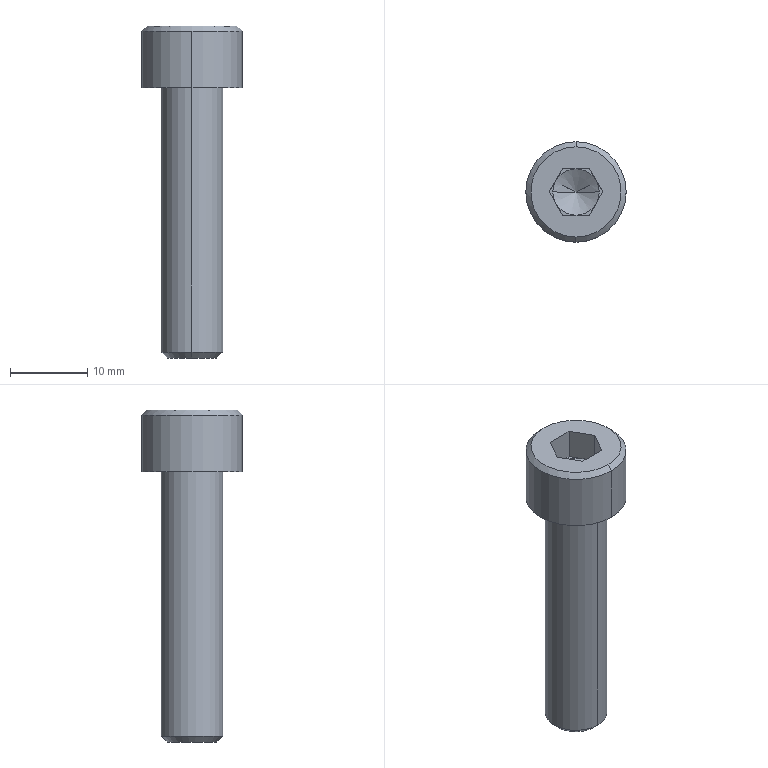Component | SolidWorks | ScrewM8-L35AndSpringWasherAssembly-2_HexSocketHeadCapScrewTAC01-M8-L35(YIHEDA)-1 | 1 solid | 25 faces | box 13 x 13 x 43 mm | volume 2665 mm3 | plane 15 | cone 6 | cylinder 4 | commonest cylinder face diameters 13 x2 8 x2
STEP:
#1=COLOUR_RGB('',0.7922,0.8196,0.9333);
#2=FILL_AREA_STYLE_COLOUR('',#1);
#3=FILL_AREA_STYLE('',(#2));
#4=SURFACE_STYLE_FILL_AREA(#3);
#5=SURFACE_SIDE_STYLE('',(#4));
#6=SURFACE_STYLE_USAGE(.BOTH.,#5);
#7=PRESENTATION_STYLE_ASSIGNMENT((#6));
#8=CARTESIAN_POINT('',(1.489,1.476,0.9883));
#9=VERTEX_POINT('',#8);
#10=CARTESIAN_POINT('',(1.489,1.222,0.9883));
#11=VERTEX_POINT('',#10);
#12=CARTESIAN_POINT('',(1.489,1.349,0.9883));
#13=DIRECTION('',(0.,0.,-1.));
#14=DIRECTION('',(0.,1.,0.));
#15=AXIS2_PLACEMENT_3D('',#12,#13,#14);
#16=CIRCLE('',#15,0.1273);
#17=EDGE_CURVE('',#9,#11,#16,.T.);
#18=ORIENTED_EDGE('',*,*,#17,.F.);
#19=CARTESIAN_POINT('',(1.489,1.507,1.019));
#20=VERTEX_POINT('',#19);
#21=CARTESIAN_POINT('',(1.489,1.507,1.019));
#22=DIRECTION('',(0.,0.7071,0.7071));
#23=VECTOR('',#22,39.37);
#24=LINE('',#21,#23);
#25=EDGE_CURVE('',#9,#20,#24,.T.);
#26=ORIENTED_EDGE('',*,*,#25,.T.);
#27=CARTESIAN_POINT('',(1.489,1.192,1.019));
#28=VERTEX_POINT('',#27);
#29=CARTESIAN_POINT('',(1.489,1.349,1.019));
#30=DIRECTION('',(0.,0.,-1.));
#31=DIRECTION('',(0.,1.,0.));
#32=AXIS2_PLACEMENT_3D('',#29,#30,#31);
#33=CIRCLE('',#32,0.1575);
#34=EDGE_CURVE('',#20,#28,#33,.T.);
#35=ORIENTED_EDGE('',*,*,#34,.T.);
#36=CARTESIAN_POINT('',(1.489,1.192,1.019));
#37=DIRECTION('',(-0.,-0.7071,0.7071));
#38=VECTOR('',#37,39.37);
#39=LINE('',#36,#38);
#40=EDGE_CURVE('',#11,#28,#39,.T.);
#41=ORIENTED_EDGE('',*,*,#40,.F.);
#42=EDGE_LOOP('',(#18,#26,#35,#41));
#43=FACE_OUTER_BOUND('',#42,.T.);
#44=CARTESIAN_POINT('',(1.489,1.349,1.019));
#45=DIRECTION('',(0.,0.,1.));
#46=DIRECTION('',(-0.,-1.,0.));
#47=AXIS2_PLACEMENT_3D('',#44,#45,#46);
#48=CONICAL_SURFACE('',#47,0.1575,0.7854);
#49=ADVANCED_FACE('',(#43),#48,.T.);
#50=CARTESIAN_POINT('',(1.489,1.579,2.681));
#51=VERTEX_POINT('',#50);
#52=CARTESIAN_POINT('',(1.489,1.119,2.681));
#53=VERTEX_POINT('',#52);
#54=CARTESIAN_POINT('',(1.489,1.349,2.681));
#55=DIRECTION('',(0.,0.,-1.));
#56=DIRECTION('',(0.,1.,0.));
#57=AXIS2_PLACEMENT_3D('',#54,#55,#56);
#58=CIRCLE('',#57,0.2303);
#59=EDGE_CURVE('',#51,#53,#58,.T.);
#60=ORIENTED_EDGE('',*,*,#59,.T.);
#61=CARTESIAN_POINT('',(1.489,1.093,2.656));
#62=VERTEX_POINT('',#61);
#63=CARTESIAN_POINT('',(1.489,1.119,2.681));
#64=DIRECTION('',(-0.,-0.7071,-0.7071));
#65=VECTOR('',#64,39.37);
#66=LINE('',#63,#65);
#67=EDGE_CURVE('',#53,#62,#66,.T.);
#68=ORIENTED_EDGE('',*,*,#67,.T.);
#69=CARTESIAN_POINT('',(1.489,1.605,2.656));
#70=VERTEX_POINT('',#69);
#71=CARTESIAN_POINT('',(1.489,1.349,2.656));
#72=DIRECTION('',(0.,0.,-1.));
#73=DIRECTION('',(0.,1.,0.));
#74=AXIS2_PLACEMENT_3D('',#71,#72,#73);
#75=CIRCLE('',#74,0.2559);
#76=EDGE_CURVE('',#70,#62,#75,.T.);
#77=ORIENTED_EDGE('',*,*,#76,.F.);
#78=CARTESIAN_POINT('',(1.489,1.579,2.681));
#79=DIRECTION('',(0.,0.7071,-0.7071));
#80=VECTOR('',#79,39.37);
#81=LINE('',#78,#80);
#82=EDGE_CURVE('',#51,#70,#81,.T.);
#83=ORIENTED_EDGE('',*,*,#82,.F.);
#84=EDGE_LOOP('',(#60,#68,#77,#83));
#85=FACE_OUTER_BOUND('',#84,.T.);
#86=CARTESIAN_POINT('',(1.489,1.349,2.681));
#87=DIRECTION('',(0.,0.,-1.));
#88=DIRECTION('',(0.,1.,0.));
#89=AXIS2_PLACEMENT_3D('',#86,#87,#88);
#90=CONICAL_SURFACE('',#89,0.2303,0.7854);
#91=ADVANCED_FACE('',(#85),#90,.T.);
#92=CARTESIAN_POINT('',(1.489,1.093,2.366));
#93=VERTEX_POINT('',#92);
#94=CARTESIAN_POINT('',(1.489,1.605,2.366));
#95=VERTEX_POINT('',#94);
#96=CARTESIAN_POINT('',(1.489,1.349,2.366));
#97=DIRECTION('',(0.,0.,-1.));
#98=DIRECTION('',(0.,1.,0.));
#99=AXIS2_PLACEMENT_3D('',#96,#97,#98);
#100=CIRCLE('',#99,0.2559);
#101=EDGE_CURVE('',#93,#95,#100,.T.);
#102=ORIENTED_EDGE('',*,*,#101,.F.);
#103=CARTESIAN_POINT('',(1.489,1.093,2.366));
#104=DIRECTION('',(0.,0.,1.));
#105=VECTOR('',#104,39.37);
#106=LINE('',#103,#105);
#107=EDGE_CURVE('',#93,#62,#106,.T.);
#108=ORIENTED_EDGE('',*,*,#107,.T.);
#109=CARTESIAN_POINT('',(1.489,1.349,2.656));
#110=DIRECTION('',(0.,0.,-1.));
#111=DIRECTION('',(0.,1.,0.));
#112=AXIS2_PLACEMENT_3D('',#109,#110,#111);
#113=CIRCLE('',#112,0.2559);
#114=EDGE_CURVE('',#62,#70,#113,.T.);
#115=ORIENTED_EDGE('',*,*,#114,.T.);
#116=CARTESIAN_POINT('',(1.489,1.605,2.366));
#117=DIRECTION('',(0.,0.,1.));
#118=VECTOR('',#117,39.37);
#119=LINE('',#116,#118);
#120=EDGE_CURVE('',#95,#70,#119,.T.);
#121=ORIENTED_EDGE('',*,*,#120,.F.);
#122=EDGE_LOOP('',(#102,#108,#115,#121));
#123=FACE_OUTER_BOUND('',#122,.T.);
#124=CARTESIAN_POINT('',(1.489,1.349,2.366));
#125=DIRECTION('',(0.,0.,1.));
#126=DIRECTION('',(0.,1.,0.));
#127=AXIS2_PLACEMENT_3D('',#124,#125,#126);
#128=CYLINDRICAL_SURFACE('',#127,0.2559);
#129=ADVANCED_FACE('',(#123),#128,.T.);
#130=CARTESIAN_POINT('',(1.489,1.349,2.456));
#131=VERTEX_POINT('',#130);
#132=CARTESIAN_POINT('',(1.371,1.349,2.524));
#133=VERTEX_POINT('',#132);
#134=CARTESIAN_POINT('',(1.371,1.349,2.524));
#135=DIRECTION('',(-0.866,0.,0.5));
#136=VECTOR('',#135,39.37);
#137=LINE('',#134,#136);
#138=EDGE_CURVE('',#131,#133,#137,.T.);
#139=ORIENTED_EDGE('',*,*,#138,.F.);
#140=CARTESIAN_POINT('',(1.607,1.349,2.524));
#141=VERTEX_POINT('',#140);
#142=CARTESIAN_POINT('',(1.607,1.349,2.524));
#143=DIRECTION('',(0.866,-0.,0.5));
#144=VECTOR('',#143,39.37);
#145=LINE('',#142,#144);
#146=EDGE_CURVE('',#131,#141,#145,.T.);
#147=ORIENTED_EDGE('',*,*,#146,.T.);
#148=CARTESIAN_POINT('',(1.592,1.408,2.524));
#149=VERTEX_POINT('',#148);
#150=CARTESIAN_POINT('',(1.489,1.349,2.524));
#151=DIRECTION('',(0.,0.,-1.));
#152=DIRECTION('',(-0.,-1.,0.));
#153=AXIS2_PLACEMENT_3D('',#150,#151,#152);
#154=CIRCLE('',#153,0.1181);
#155=EDGE_CURVE('',#149,#141,#154,.T.);
#156=ORIENTED_EDGE('',*,*,#155,.F.);
#157=CARTESIAN_POINT('',(1.489,1.467,2.524));
#158=VERTEX_POINT('',#157);
#159=CARTESIAN_POINT('',(1.489,1.349,2.524));
#160=DIRECTION('',(0.,0.,-1.));
#161=DIRECTION('',(-0.,-1.,0.));
#162=AXIS2_PLACEMENT_3D('',#159,#160,#161);
#163=CIRCLE('',#162,0.1181);
#164=EDGE_CURVE('',#158,#149,#163,.T.);
#165=ORIENTED_EDGE('',*,*,#164,.F.);
#166=CARTESIAN_POINT('',(1.387,1.408,2.524));
#167=VERTEX_POINT('',#166);
#168=CARTESIAN_POINT('',(1.489,1.349,2.524));
#169=DIRECTION('',(0.,0.,-1.));
#170=DIRECTION('',(-0.,-1.,0.));
#171=AXIS2_PLACEMENT_3D('',#168,#169,#170);
#172=CIRCLE('',#171,0.1181);
#173=EDGE_CURVE('',#167,#158,#172,.T.);
#174=ORIENTED_EDGE('',*,*,#173,.F.);
#175=CARTESIAN_POINT('',(1.489,1.349,2.524));
#176=DIRECTION('',(0.,0.,-1.));
#177=DIRECTION('',(-0.,-1.,0.));
#178=AXIS2_PLACEMENT_3D('',#175,#176,#177);
#179=CIRCLE('',#178,0.1181);
#180=EDGE_CURVE('',#133,#167,#179,.T.);
#181=ORIENTED_EDGE('',*,*,#180,.F.);
#182=EDGE_LOOP('',(#139,#147,#156,#165,#174,#181));
#183=FACE_OUTER_BOUND('',#182,.T.);
#184=CARTESIAN_POINT('',(1.489,1.349,2.524));
#185=DIRECTION('',(0.,-0.,1.));
#186=DIRECTION('',(-1.,0.,0.));
#187=AXIS2_PLACEMENT_3D('',#184,#185,#186);
#188=CONICAL_SURFACE('',#187,0.1181,1.047);
#189=ADVANCED_FACE('',(#183),#188,.F.);
#190=CARTESIAN_POINT('',(1.489,1.349,1.019));
#191=DIRECTION('',(0.,0.,-1.));
#192=DIRECTION('',(0.,1.,0.));
#193=AXIS2_PLACEMENT_3D('',#190,#191,#192);
#194=CIRCLE('',#193,0.1575);
#195=EDGE_CURVE('',#28,#20,#194,.T.);
#196=ORIENTED_EDGE('',*,*,#195,.F.);
#197=CARTESIAN_POINT('',(1.489,1.192,2.366));
#198=VERTEX_POINT('',#197);
#199=CARTESIAN_POINT('',(1.489,1.192,0.9883));
#200=DIRECTION('',(0.,0.,1.));
#201=VECTOR('',#200,39.37);
#202=LINE('',#199,#201);
#203=EDGE_CURVE('',#28,#198,#202,.T.);
#204=ORIENTED_EDGE('',*,*,#203,.T.);
#205=CARTESIAN_POINT('',(1.489,1.507,2.366));
#206=VERTEX_POINT('',#205);
#207=CARTESIAN_POINT('',(1.489,1.349,2.366));
#208=DIRECTION('',(0.,0.,-1.));
#209=DIRECTION('',(0.,1.,0.));
#210=AXIS2_PLACEMENT_3D('',#207,#208,#209);
#211=CIRCLE('',#210,0.1575);
#212=EDGE_CURVE('',#198,#206,#211,.T.);
#213=ORIENTED_EDGE('',*,*,#212,.T.);
#214=CARTESIAN_POINT('',(1.489,1.507,0.9883));
#215=DIRECTION('',(0.,0.,1.));
#216=VECTOR('',#215,39.37);
#217=LINE('',#214,#216);
#218=EDGE_CURVE('',#20,#206,#217,.T.);
#219=ORIENTED_EDGE('',*,*,#218,.F.);
#220=EDGE_LOOP('',(#196,#204,#213,#219));
#221=FACE_OUTER_BOUND('',#220,.T.);
#222=CARTESIAN_POINT('',(1.489,1.349,0.9883));
#223=DIRECTION('',(0.,0.,1.));
#224=DIRECTION('',(0.,1.,0.));
#225=AXIS2_PLACEMENT_3D('',#222,#223,#224);
#226=CYLINDRICAL_SURFACE('',#225,0.1575);
#227=ADVANCED_FACE('',(#221),#226,.T.);
#228=CARTESIAN_POINT('',(1.353,1.349,2.524));
#229=VERTEX_POINT('',#228);
#230=CARTESIAN_POINT('',(1.387,1.29,2.524));
#231=VERTEX_POINT('',#230);
#232=CARTESIAN_POINT('',(1.353,1.349,2.524));
#233=DIRECTION('',(0.5,-0.866,0.));
#234=VECTOR('',#233,39.37);
#235=LINE('',#232,#234);
#236=EDGE_CURVE('',#229,#231,#235,.T.);
#237=ORIENTED_EDGE('',*,*,#236,.T.);
#238=CARTESIAN_POINT('',(1.489,1.349,2.524));
#239=DIRECTION('',(0.,0.,-1.));
#240=DIRECTION('',(-0.,-1.,0.));
#241=AXIS2_PLACEMENT_3D('',#238,#239,#240);
#242=CIRCLE('',#241,0.1181);
#243=EDGE_CURVE('',#231,#133,#242,.T.);
#244=ORIENTED_EDGE('',*,*,#243,.T.);
#245=ORIENTED_EDGE('',*,*,#180,.T.);
#246=CARTESIAN_POINT('',(1.421,1.467,2.524));
#247=DIRECTION('',(-0.5,-0.866,0.));
#248=VECTOR('',#247,39.37);
#249=LINE('',#246,#248);
#250=EDGE_CURVE('',#167,#229,#249,.T.);
#251=ORIENTED_EDGE('',*,*,#250,.T.);
#252=EDGE_LOOP('',(#237,#244,#245,#251));
#253=FACE_OUTER_BOUND('',#252,.T.);
#254=CARTESIAN_POINT('',(1.489,1.349,2.524));
#255=DIRECTION('',(0.,0.,1.));
#256=DIRECTION('',(-0.,-1.,0.));
#257=AXIS2_PLACEMENT_3D('',#254,#255,#256);
#258=PLANE('',#257);
#259=ADVANCED_FACE('',(#253),#258,.T.);
#260=ORIENTED_EDGE('',*,*,#203,.F.);
#261=ORIENTED_EDGE('',*,*,#34,.F.);
#262=ORIENTED_EDGE('',*,*,#218,.T.);
#263=CARTESIAN_POINT('',(1.489,1.349,2.366));
#264=DIRECTION('',(0.,0.,-1.));
#265=DIRECTION('',(0.,1.,0.));
#266=AXIS2_PLACEMENT_3D('',#263,#264,#265);
#267=CIRCLE('',#266,0.1575);
#268=EDGE_CURVE('',#206,#198,#267,.T.);
#269=ORIENTED_EDGE('',*,*,#268,.T.);
#270=EDGE_LOOP('',(#260,#261,#262,#269));
#271=FACE_OUTER_BOUND('',#270,.T.);
#272=CARTESIAN_POINT('',(1.489,1.349,0.9883));
#273=DIRECTION('',(0.,0.,1.));
#274=DIRECTION('',(0.,1.,0.));
#275=AXIS2_PLACEMENT_3D('',#272,#273,#274);
#276=CYLINDRICAL_SURFACE('',#275,0.1575);
#277=ADVANCED_FACE('',(#271),#276,.T.);
#278=ORIENTED_EDGE('',*,*,#146,.F.);
#279=ORIENTED_EDGE('',*,*,#138,.T.);
#280=ORIENTED_EDGE('',*,*,#243,.F.);
#281=CARTESIAN_POINT('',(1.489,1.231,2.524));
#282=VERTEX_POINT('',#281);
#283=CARTESIAN_POINT('',(1.489,1.349,2.524));
#284=DIRECTION('',(0.,0.,-1.));
#285=DIRECTION('',(-0.,-1.,0.));
#286=AXIS2_PLACEMENT_3D('',#283,#284,#285);
#287=CIRCLE('',#286,0.1181);
#288=EDGE_CURVE('',#282,#231,#287,.T.);
#289=ORIENTED_EDGE('',*,*,#288,.F.);
#290=CARTESIAN_POINT('',(1.592,1.29,2.524));
#291=VERTEX_POINT('',#290);
#292=CARTESIAN_POINT('',(1.489,1.349,2.524));
#293=DIRECTION('',(0.,0.,-1.));
#294=DIRECTION('',(-0.,-1.,0.));
#295=AXIS2_PLACEMENT_3D('',#292,#293,#294);
#296=CIRCLE('',#295,0.1181);
#297=EDGE_CURVE('',#291,#282,#296,.T.);
#298=ORIENTED_EDGE('',*,*,#297,.F.);
#299=CARTESIAN_POINT('',(1.489,1.349,2.524));
#300=DIRECTION('',(0.,0.,-1.));
#301=DIRECTION('',(-0.,-1.,0.));
#302=AXIS2_PLACEMENT_3D('',#299,#300,#301);
#303=CIRCLE('',#302,0.1181);
#304=EDGE_CURVE('',#141,#291,#303,.T.);
#305=ORIENTED_EDGE('',*,*,#304,.F.);
#306=EDGE_LOOP('',(#278,#279,#280,#289,#298,#305));
#307=FACE_OUTER_BOUND('',#306,.T.);
#308=CARTESIAN_POINT('',(1.489,1.349,2.524));
#309=DIRECTION('',(0.,-0.,1.));
#310=DIRECTION('',(-1.,0.,0.));
#311=AXIS2_PLACEMENT_3D('',#308,#309,#310);
#312=CONICAL_SURFACE('',#311,0.1181,1.047);
#313=ADVANCED_FACE('',(#307),#312,.F.);
#314=CARTESIAN_POINT('',(1.558,1.467,2.681));
#315=VERTEX_POINT('',#314);
#316=CARTESIAN_POINT('',(1.421,1.467,2.681));
#317=VERTEX_POINT('',#316);
#318=CARTESIAN_POINT('',(1.558,1.467,2.681));
#319=DIRECTION('',(-1.,0.,0.));
#320=VECTOR('',#319,39.37);
#321=LINE('',#318,#320);
#322=EDGE_CURVE('',#315,#317,#321,.T.);
#323=ORIENTED_EDGE('',*,*,#322,.T.);
#324=CARTESIAN_POINT('',(1.421,1.467,2.524));
#325=VERTEX_POINT('',#324);
#326=CARTESIAN_POINT('',(1.421,1.467,2.524));
#327=DIRECTION('',(0.,0.,1.));
#328=VECTOR('',#327,39.37);
#329=LINE('',#326,#328);
#330=EDGE_CURVE('',#325,#317,#329,.T.);
#331=ORIENTED_EDGE('',*,*,#330,.F.);
#332=CARTESIAN_POINT('',(1.558,1.467,2.524));
#333=DIRECTION('',(-1.,0.,0.));
#334=VECTOR('',#333,39.37);
#335=LINE('',#332,#334);
#336=EDGE_CURVE('',#158,#325,#335,.T.);
#337=ORIENTED_EDGE('',*,*,#336,.F.);
#338=CARTESIAN_POINT('',(1.558,1.467,2.524));
#339=VERTEX_POINT('',#338);
#340=CARTESIAN_POINT('',(1.558,1.467,2.524));
#341=DIRECTION('',(-1.,0.,0.));
#342=VECTOR('',#341,39.37);
#343=LINE('',#340,#342);
#344=EDGE_CURVE('',#339,#158,#343,.T.);
#345=ORIENTED_EDGE('',*,*,#344,.F.);
#346=CARTESIAN_POINT('',(1.558,1.467,2.524));
#347=DIRECTION('',(0.,0.,1.));
#348=VECTOR('',#347,39.37);
#349=LINE('',#346,#348);
#350=EDGE_CURVE('',#339,#315,#349,.T.);
#351=ORIENTED_EDGE('',*,*,#350,.T.);
#352=EDGE_LOOP('',(#323,#331,#337,#345,#351));
#353=FACE_OUTER_BOUND('',#352,.T.);
#354=CARTESIAN_POINT('',(1.558,1.467,2.524));
#355=DIRECTION('',(0.,1.,0.));
#356=DIRECTION('',(0.,0.,1.));
#357=AXIS2_PLACEMENT_3D('',#354,#355,#356);
#358=PLANE('',#357);
#359=ADVANCED_FACE('',(#353),#358,.F.);
#360=CARTESIAN_POINT('',(1.558,1.231,2.681));
#361=VERTEX_POINT('',#360);
#362=CARTESIAN_POINT('',(1.626,1.349,2.681));
#363=VERTEX_POINT('',#362);
#364=CARTESIAN_POINT('',(1.558,1.231,2.681));
#365=DIRECTION('',(0.5,0.866,0.));
#366=VECTOR('',#365,39.37);
#367=LINE('',#364,#366);
#368=EDGE_CURVE('',#361,#363,#367,.T.);
#369=ORIENTED_EDGE('',*,*,#368,.T.);
#370=CARTESIAN_POINT('',(1.626,1.349,2.524));
#371=VERTEX_POINT('',#370);
#372=CARTESIAN_POINT('',(1.626,1.349,2.524));
#373=DIRECTION('',(0.,0.,1.));
#374=VECTOR('',#373,39.37);
#375=LINE('',#372,#374);
#376=EDGE_CURVE('',#371,#363,#375,.T.);
#377=ORIENTED_EDGE('',*,*,#376,.F.);
#378=CARTESIAN_POINT('',(1.558,1.231,2.524));
#379=DIRECTION('',(0.5,0.866,0.));
#380=VECTOR('',#379,39.37);
#381=LINE('',#378,#380);
#382=EDGE_CURVE('',#291,#371,#381,.T.);
#383=ORIENTED_EDGE('',*,*,#382,.F.);
#384=CARTESIAN_POINT('',(1.558,1.231,2.524));
#385=VERTEX_POINT('',#384);
#386=CARTESIAN_POINT('',(1.558,1.231,2.524));
#387=DIRECTION('',(0.5,0.866,0.));
#388=VECTOR('',#387,39.37);
#389=LINE('',#386,#388);
#390=EDGE_CURVE('',#385,#291,#389,.T.);
#391=ORIENTED_EDGE('',*,*,#390,.F.);
#392=CARTESIAN_POINT('',(1.558,1.231,2.524));
#393=DIRECTION('',(0.,0.,1.));
#394=VECTOR('',#393,39.37);
#395=LINE('',#392,#394);
#396=EDGE_CURVE('',#385,#361,#395,.T.);
#397=ORIENTED_EDGE('',*,*,#396,.T.);
#398=EDGE_LOOP('',(#369,#377,#383,#391,#397));
#399=FACE_OUTER_BOUND('',#398,.T.);
#400=CARTESIAN_POINT('',(1.558,1.231,2.524));
#401=DIRECTION('',(0.866,-0.5,0.));
#402=DIRECTION('',(0.,0.,-1.));
#403=AXIS2_PLACEMENT_3D('',#400,#401,#402);
#404=PLANE('',#403);
#405=ADVANCED_FACE('',(#399),#404,.F.);
#406=ORIENTED_EDGE('',*,*,#390,.T.);
#407=ORIENTED_EDGE('',*,*,#297,.T.);
#408=CARTESIAN_POINT('',(1.421,1.231,2.524));
#409=DIRECTION('',(1.,-0.,0.));
#410=VECTOR('',#409,39.37);
#411=LINE('',#408,#410);
#412=EDGE_CURVE('',#282,#385,#411,.T.);
#413=ORIENTED_EDGE('',*,*,#412,.T.);
#414=EDGE_LOOP('',(#406,#407,#413));
#415=FACE_OUTER_BOUND('',#414,.T.);
#416=CARTESIAN_POINT('',(1.489,1.349,2.524));
#417=DIRECTION('',(0.,0.,1.));
#418=DIRECTION('',(-0.,-1.,0.));
#419=AXIS2_PLACEMENT_3D('',#416,#417,#418);
#420=PLANE('',#419);
#421=ADVANCED_FACE('',(#415),#420,.T.);
#422=CARTESIAN_POINT('',(1.489,1.349,2.366));
#423=DIRECTION('',(0.,0.,-1.));
#424=DIRECTION('',(0.,1.,0.));
#425=AXIS2_PLACEMENT_3D('',#422,#423,#424);
#426=CIRCLE('',#425,0.2559);
#427=EDGE_CURVE('',#95,#93,#426,.T.);
#428=ORIENTED_EDGE('',*,*,#427,.T.);
#429=ORIENTED_EDGE('',*,*,#101,.T.);
#430=EDGE_LOOP('',(#428,#429));
#431=FACE_OUTER_BOUND('',#430,.T.);
#432=ORIENTED_EDGE('',*,*,#268,.F.);
#433=ORIENTED_EDGE('',*,*,#212,.F.);
#434=EDGE_LOOP('',(#432,#433));
#435=FACE_BOUND('',#434,.T.);
#436=CARTESIAN_POINT('',(1.745,1.349,2.366));
#437=DIRECTION('',(0.,0.,1.));
#438=DIRECTION('',(-0.,-1.,0.));
#439=AXIS2_PLACEMENT_3D('',#436,#437,#438);
#440=PLANE('',#439);
#441=ADVANCED_FACE('',(#431,#435),#440,.F.);
#442=ORIENTED_EDGE('',*,*,#59,.F.);
#443=CARTESIAN_POINT('',(1.489,1.349,2.681));
#444=DIRECTION('',(0.,0.,-1.));
#445=DIRECTION('',(0.,1.,0.));
#446=AXIS2_PLACEMENT_3D('',#443,#444,#445);
#447=CIRCLE('',#446,0.2303);
#448=EDGE_CURVE('',#53,#51,#447,.T.);
#449=ORIENTED_EDGE('',*,*,#448,.F.);
#450=EDGE_LOOP('',(#442,#449));
#451=FACE_OUTER_BOUND('',#450,.T.);
#452=CARTESIAN_POINT('',(1.353,1.349,2.681));
#453=VERTEX_POINT('',#452);
#454=CARTESIAN_POINT('',(1.421,1.231,2.681));
#455=VERTEX_POINT('',#454);
#456=CARTESIAN_POINT('',(1.353,1.349,2.681));
#457=DIRECTION('',(0.5,-0.866,0.));
#458=VECTOR('',#457,39.37);
#459=LINE('',#456,#458);
#460=EDGE_CURVE('',#453,#455,#459,.T.);
#461=ORIENTED_EDGE('',*,*,#460,.F.);
#462=CARTESIAN_POINT('',(1.421,1.467,2.681));
#463=DIRECTION('',(-0.5,-0.866,0.));
#464=VECTOR('',#463,39.37);
#465=LINE('',#462,#464);
#466=EDGE_CURVE('',#317,#453,#465,.T.);
#467=ORIENTED_EDGE('',*,*,#466,.F.);
#468=ORIENTED_EDGE('',*,*,#322,.F.);
#469=CARTESIAN_POINT('',(1.626,1.349,2.681));
#470=DIRECTION('',(-0.5,0.866,0.));
#471=VECTOR('',#470,39.37);
#472=LINE('',#469,#471);
#473=EDGE_CURVE('',#363,#315,#472,.T.);
#474=ORIENTED_EDGE('',*,*,#473,.F.);
#475=ORIENTED_EDGE('',*,*,#368,.F.);
#476=CARTESIAN_POINT('',(1.421,1.231,2.681));
#477=DIRECTION('',(1.,-0.,0.));
#478=VECTOR('',#477,39.37);
#479=LINE('',#476,#478);
#480=EDGE_CURVE('',#455,#361,#479,.T.);
#481=ORIENTED_EDGE('',*,*,#480,.F.);
#482=EDGE_LOOP('',(#461,#467,#468,#474,#475,#481));
#483=FACE_BOUND('',#482,.T.);
#484=CARTESIAN_POINT('',(1.489,1.349,2.681));
#485=DIRECTION('',(0.,0.,-1.));
#486=DIRECTION('',(-1.,0.,0.));
#487=AXIS2_PLACEMENT_3D('',#484,#485,#486);
#488=PLANE('',#487);
#489=ADVANCED_FACE('',(#451,#483),#488,.F.);
#490=CARTESIAN_POINT('',(1.489,1.349,0.9883));
#491=DIRECTION('',(0.,0.,-1.));
#492=DIRECTION('',(0.,1.,0.));
#493=AXIS2_PLACEMENT_3D('',#490,#491,#492);
#494=CIRCLE('',#493,0.1273);
#495=EDGE_CURVE('',#11,#9,#494,.T.);
#496=ORIENTED_EDGE('',*,*,#495,.T.);
#497=ORIENTED_EDGE('',*,*,#17,.T.);
#498=EDGE_LOOP('',(#496,#497));
#499=FACE_OUTER_BOUND('',#498,.T.);
#500=CARTESIAN_POINT('',(1.617,1.349,0.9883));
#501=DIRECTION('',(0.,0.,1.));
#502=DIRECTION('',(-0.,-1.,0.));
#503=AXIS2_PLACEMENT_3D('',#500,#501,#502);
#504=PLANE('',#503);
#505=ADVANCED_FACE('',(#499),#504,.F.);
#506=ORIENTED_EDGE('',*,*,#107,.F.);
#507=ORIENTED_EDGE('',*,*,#427,.F.);
#508=ORIENTED_EDGE('',*,*,#120,.T.);
#509=ORIENTED_EDGE('',*,*,#76,.T.);
#510=EDGE_LOOP('',(#506,#507,#508,#509));
#511=FACE_OUTER_BOUND('',#510,.T.);
#512=CARTESIAN_POINT('',(1.489,1.349,2.366));
#513=DIRECTION('',(0.,0.,1.));
#514=DIRECTION('',(0.,1.,0.));
#515=AXIS2_PLACEMENT_3D('',#512,#513,#514);
#516=CYLINDRICAL_SURFACE('',#515,0.2559);
#517=ADVANCED_FACE('',(#511),#516,.T.);
#518=ORIENTED_EDGE('',*,*,#466,.T.);
#519=CARTESIAN_POINT('',(1.353,1.349,2.524));
#520=DIRECTION('',(0.,0.,1.));
#521=VECTOR('',#520,39.37);
#522=LINE('',#519,#521);
#523=EDGE_CURVE('',#229,#453,#522,.T.);
#524=ORIENTED_EDGE('',*,*,#523,.F.);
#525=ORIENTED_EDGE('',*,*,#250,.F.);
#526=CARTESIAN_POINT('',(1.421,1.467,2.524));
#527=DIRECTION('',(-0.5,-0.866,0.));
#528=VECTOR('',#527,39.37);
#529=LINE('',#526,#528);
#530=EDGE_CURVE('',#325,#167,#529,.T.);
#531=ORIENTED_EDGE('',*,*,#530,.F.);
#532=ORIENTED_EDGE('',*,*,#330,.T.);
#533=EDGE_LOOP('',(#518,#524,#525,#531,#532));
#534=FACE_OUTER_BOUND('',#533,.T.);
#535=CARTESIAN_POINT('',(1.421,1.467,2.524));
#536=DIRECTION('',(-0.866,0.5,0.));
#537=DIRECTION('',(0.5,0.866,0.));
#538=AXIS2_PLACEMENT_3D('',#535,#536,#537);
#539=PLANE('',#538);
#540=ADVANCED_FACE('',(#534),#539,.F.);
#541=ORIENTED_EDGE('',*,*,#67,.F.);
#542=ORIENTED_EDGE('',*,*,#448,.T.);
#543=ORIENTED_EDGE('',*,*,#82,.T.);
#544=ORIENTED_EDGE('',*,*,#114,.F.);
#545=EDGE_LOOP('',(#541,#542,#543,#544));
#546=FACE_OUTER_BOUND('',#545,.T.);
#547=CARTESIAN_POINT('',(1.489,1.349,2.681));
#548=DIRECTION('',(0.,0.,-1.));
#549=DIRECTION('',(0.,1.,0.));
#550=AXIS2_PLACEMENT_3D('',#547,#548,#549);
#551=CONICAL_SURFACE('',#550,0.2303,0.7854);
#552=ADVANCED_FACE('',(#546),#551,.T.);
#553=ORIENTED_EDGE('',*,*,#460,.T.);
#554=CARTESIAN_POINT('',(1.421,1.231,2.524));
#555=VERTEX_POINT('',#554);
#556=CARTESIAN_POINT('',(1.421,1.231,2.524));
#557=DIRECTION('',(0.,0.,1.));
#558=VECTOR('',#557,39.37);
#559=LINE('',#556,#558);
#560=EDGE_CURVE('',#555,#455,#559,.T.);
#561=ORIENTED_EDGE('',*,*,#560,.F.);
#562=CARTESIAN_POINT('',(1.353,1.349,2.524));
#563=DIRECTION('',(0.5,-0.866,0.));
#564=VECTOR('',#563,39.37);
#565=LINE('',#562,#564);
#566=EDGE_CURVE('',#231,#555,#565,.T.);
#567=ORIENTED_EDGE('',*,*,#566,.F.);
#568=ORIENTED_EDGE('',*,*,#236,.F.);
#569=ORIENTED_EDGE('',*,*,#523,.T.);
#570=EDGE_LOOP('',(#553,#561,#567,#568,#569));
#571=FACE_OUTER_BOUND('',#570,.T.);
#572=CARTESIAN_POINT('',(1.353,1.349,2.524));
#573=DIRECTION('',(-0.866,-0.5,0.));
#574=DIRECTION('',(0.,0.,-1.));
#575=AXIS2_PLACEMENT_3D('',#572,#573,#574);
#576=PLANE('',#575);
#577=ADVANCED_FACE('',(#571),#576,.F.);
#578=ORIENTED_EDGE('',*,*,#480,.T.);
#579=ORIENTED_EDGE('',*,*,#396,.F.);
#580=ORIENTED_EDGE('',*,*,#412,.F.);
#581=CARTESIAN_POINT('',(1.421,1.231,2.524));
#582=DIRECTION('',(1.,-0.,0.));
#583=VECTOR('',#582,39.37);
#584=LINE('',#581,#583);
#585=EDGE_CURVE('',#555,#282,#584,.T.);
#586=ORIENTED_EDGE('',*,*,#585,.F.);
#587=ORIENTED_EDGE('',*,*,#560,.T.);
#588=EDGE_LOOP('',(#578,#579,#580,#586,#587));
#589=FACE_OUTER_BOUND('',#588,.T.);
#590=CARTESIAN_POINT('',(1.421,1.231,2.524));
#591=DIRECTION('',(-0.,-1.,0.));
#592=DIRECTION('',(1.,-0.,0.));
#593=AXIS2_PLACEMENT_3D('',#590,#591,#592);
#594=PLANE('',#593);
#595=ADVANCED_FACE('',(#589),#594,.F.);
#596=ORIENTED_EDGE('',*,*,#585,.T.);
#597=ORIENTED_EDGE('',*,*,#288,.T.);
#598=ORIENTED_EDGE('',*,*,#566,.T.);
#599=EDGE_LOOP('',(#596,#597,#598));
#600=FACE_OUTER_BOUND('',#599,.T.);
#601=CARTESIAN_POINT('',(1.489,1.349,2.524));
#602=DIRECTION('',(0.,0.,1.));
#603=DIRECTION('',(-0.,-1.,0.));
#604=AXIS2_PLACEMENT_3D('',#601,#602,#603);
#605=PLANE('',#604);
#606=ADVANCED_FACE('',(#600),#605,.T.);
#607=ORIENTED_EDGE('',*,*,#530,.T.);
#608=ORIENTED_EDGE('',*,*,#173,.T.);
#609=ORIENTED_EDGE('',*,*,#336,.T.);
#610=EDGE_LOOP('',(#607,#608,#609));
#611=FACE_OUTER_BOUND('',#610,.T.);
#612=CARTESIAN_POINT('',(1.489,1.349,2.524));
#613=DIRECTION('',(0.,0.,1.));
#614=DIRECTION('',(-0.,-1.,0.));
#615=AXIS2_PLACEMENT_3D('',#612,#613,#614);
#616=PLANE('',#615);
#617=ADVANCED_FACE('',(#611),#616,.T.);
#618=ORIENTED_EDGE('',*,*,#344,.T.);
#619=ORIENTED_EDGE('',*,*,#164,.T.);
#620=CARTESIAN_POINT('',(1.626,1.349,2.524));
#621=DIRECTION('',(-0.5,0.866,0.));
#622=VECTOR('',#621,39.37);
#623=LINE('',#620,#622);
#624=EDGE_CURVE('',#149,#339,#623,.T.);
#625=ORIENTED_EDGE('',*,*,#624,.T.);
#626=EDGE_LOOP('',(#618,#619,#625));
#627=FACE_OUTER_BOUND('',#626,.T.);
#628=CARTESIAN_POINT('',(1.489,1.349,2.524));
#629=DIRECTION('',(0.,0.,1.));
#630=DIRECTION('',(-0.,-1.,0.));
#631=AXIS2_PLACEMENT_3D('',#628,#629,#630);
#632=PLANE('',#631);
#633=ADVANCED_FACE('',(#627),#632,.T.);
#634=ORIENTED_EDGE('',*,*,#473,.T.);
#635=ORIENTED_EDGE('',*,*,#350,.F.);
#636=ORIENTED_EDGE('',*,*,#624,.F.);
#637=CARTESIAN_POINT('',(1.626,1.349,2.524));
#638=DIRECTION('',(-0.5,0.866,0.));
#639=VECTOR('',#638,39.37);
#640=LINE('',#637,#639);
#641=EDGE_CURVE('',#371,#149,#640,.T.);
#642=ORIENTED_EDGE('',*,*,#641,.F.);
#643=ORIENTED_EDGE('',*,*,#376,.T.);
#644=EDGE_LOOP('',(#634,#635,#636,#642,#643));
#645=FACE_OUTER_BOUND('',#644,.T.);
#646=CARTESIAN_POINT('',(1.626,1.349,2.524));
#647=DIRECTION('',(0.866,0.5,0.));
#648=DIRECTION('',(0.,0.,1.));
#649=AXIS2_PLACEMENT_3D('',#646,#647,#648);
#650=PLANE('',#649);
#651=ADVANCED_FACE('',(#645),#650,.F.);
#652=ORIENTED_EDGE('',*,*,#25,.F.);
#653=ORIENTED_EDGE('',*,*,#495,.F.);
#654=ORIENTED_EDGE('',*,*,#40,.T.);
#655=ORIENTED_EDGE('',*,*,#195,.T.);
#656=EDGE_LOOP('',(#652,#653,#654,#655));
#657=FACE_OUTER_BOUND('',#656,.T.);
#658=CARTESIAN_POINT('',(1.489,1.349,1.019));
#659=DIRECTION('',(0.,0.,1.));
#660=DIRECTION('',(-0.,-1.,0.));
#661=AXIS2_PLACEMENT_3D('',#658,#659,#660);
#662=CONICAL_SURFACE('',#661,0.1575,0.7854);
#663=ADVANCED_FACE('',(#657),#662,.T.);
#664=ORIENTED_EDGE('',*,*,#641,.T.);
#665=ORIENTED_EDGE('',*,*,#155,.T.);
#666=ORIENTED_EDGE('',*,*,#304,.T.);
#667=ORIENTED_EDGE('',*,*,#382,.T.);
#668=EDGE_LOOP('',(#664,#665,#666,#667));
#669=FACE_OUTER_BOUND('',#668,.T.);
#670=CARTESIAN_POINT('',(1.489,1.349,2.524));
#671=DIRECTION('',(0.,0.,1.));
#672=DIRECTION('',(-0.,-1.,0.));
#673=AXIS2_PLACEMENT_3D('',#670,#671,#672);
#674=PLANE('',#673);
#675=ADVANCED_FACE('',(#669),#674,.T.);
#676=CLOSED_SHELL('',(#49,#91,#129,#189,#227,#259,#277,#313,#359,#405,#421,#441,#489,#505,#517,#540,#552,#577,#595,#606,#617,#633,#651,#663,#675));
#677=MANIFOLD_SOLID_BREP('',#676);
#678=STYLED_ITEM('',(#7),#677);
#679=PRESENTATION_LAYER_ASSIGNMENT('','',(#678));
#680=CARTESIAN_POINT('',(0.,0.,0.));
#681=DIRECTION('',(0.,0.,1.));
#682=DIRECTION('',(1.,0.,0.));
#683=AXIS2_PLACEMENT_3D('',#680,#681,#682);
#684=(LENGTH_UNIT()NAMED_UNIT(*)SI_UNIT($,.METRE.));
#685=LENGTH_MEASURE_WITH_UNIT(LENGTH_MEASURE(0.0254),#684);
#686=DIMENSIONAL_EXPONENTS(1.,0.,0.,0.,0.,0.,0.);
#687=(CONVERSION_BASED_UNIT('',#685)LENGTH_UNIT()NAMED_UNIT(#686));
#688=UNCERTAINTY_MEASURE_WITH_UNIT(LENGTH_MEASURE(0.00001),#687,'','');
#689=(NAMED_UNIT(*)PLANE_ANGLE_UNIT()SI_UNIT($,.RADIAN.));
#690=(NAMED_UNIT(*)SI_UNIT($,.STERADIAN.)SOLID_ANGLE_UNIT());
#691=(GEOMETRIC_REPRESENTATION_CONTEXT(3)GLOBAL_UNCERTAINTY_ASSIGNED_CONTEXT((#688))GLOBAL_UNIT_ASSIGNED_CONTEXT((#687,#689,#690))REPRESENTATION_CONTEXT('',''));
#692=ADVANCED_BREP_SHAPE_REPRESENTATION('',(#677,#683),#691);
#693=(LENGTH_UNIT()NAMED_UNIT(*)SI_UNIT($,.METRE.));
#694=LENGTH_MEASURE_WITH_UNIT(LENGTH_MEASURE(0.0254),#693);
#695=DIMENSIONAL_EXPONENTS(1.,0.,0.,0.,0.,0.,0.);
#696=(CONVERSION_BASED_UNIT('',#694)LENGTH_UNIT()NAMED_UNIT(#695));
#697=UNCERTAINTY_MEASURE_WITH_UNIT(LENGTH_MEASURE(0.00001),#696,'','');
#698=(NAMED_UNIT(*)PLANE_ANGLE_UNIT()SI_UNIT($,.RADIAN.));
#699=(NAMED_UNIT(*)SI_UNIT($,.STERADIAN.)SOLID_ANGLE_UNIT());
#700=(GEOMETRIC_REPRESENTATION_CONTEXT(3)GLOBAL_UNCERTAINTY_ASSIGNED_CONTEXT((#697))GLOBAL_UNIT_ASSIGNED_CONTEXT((#696,#698,#699))REPRESENTATION_CONTEXT('',''));
#701=MECHANICAL_DESIGN_GEOMETRIC_PRESENTATION_REPRESENTATION('',(#678),#700);